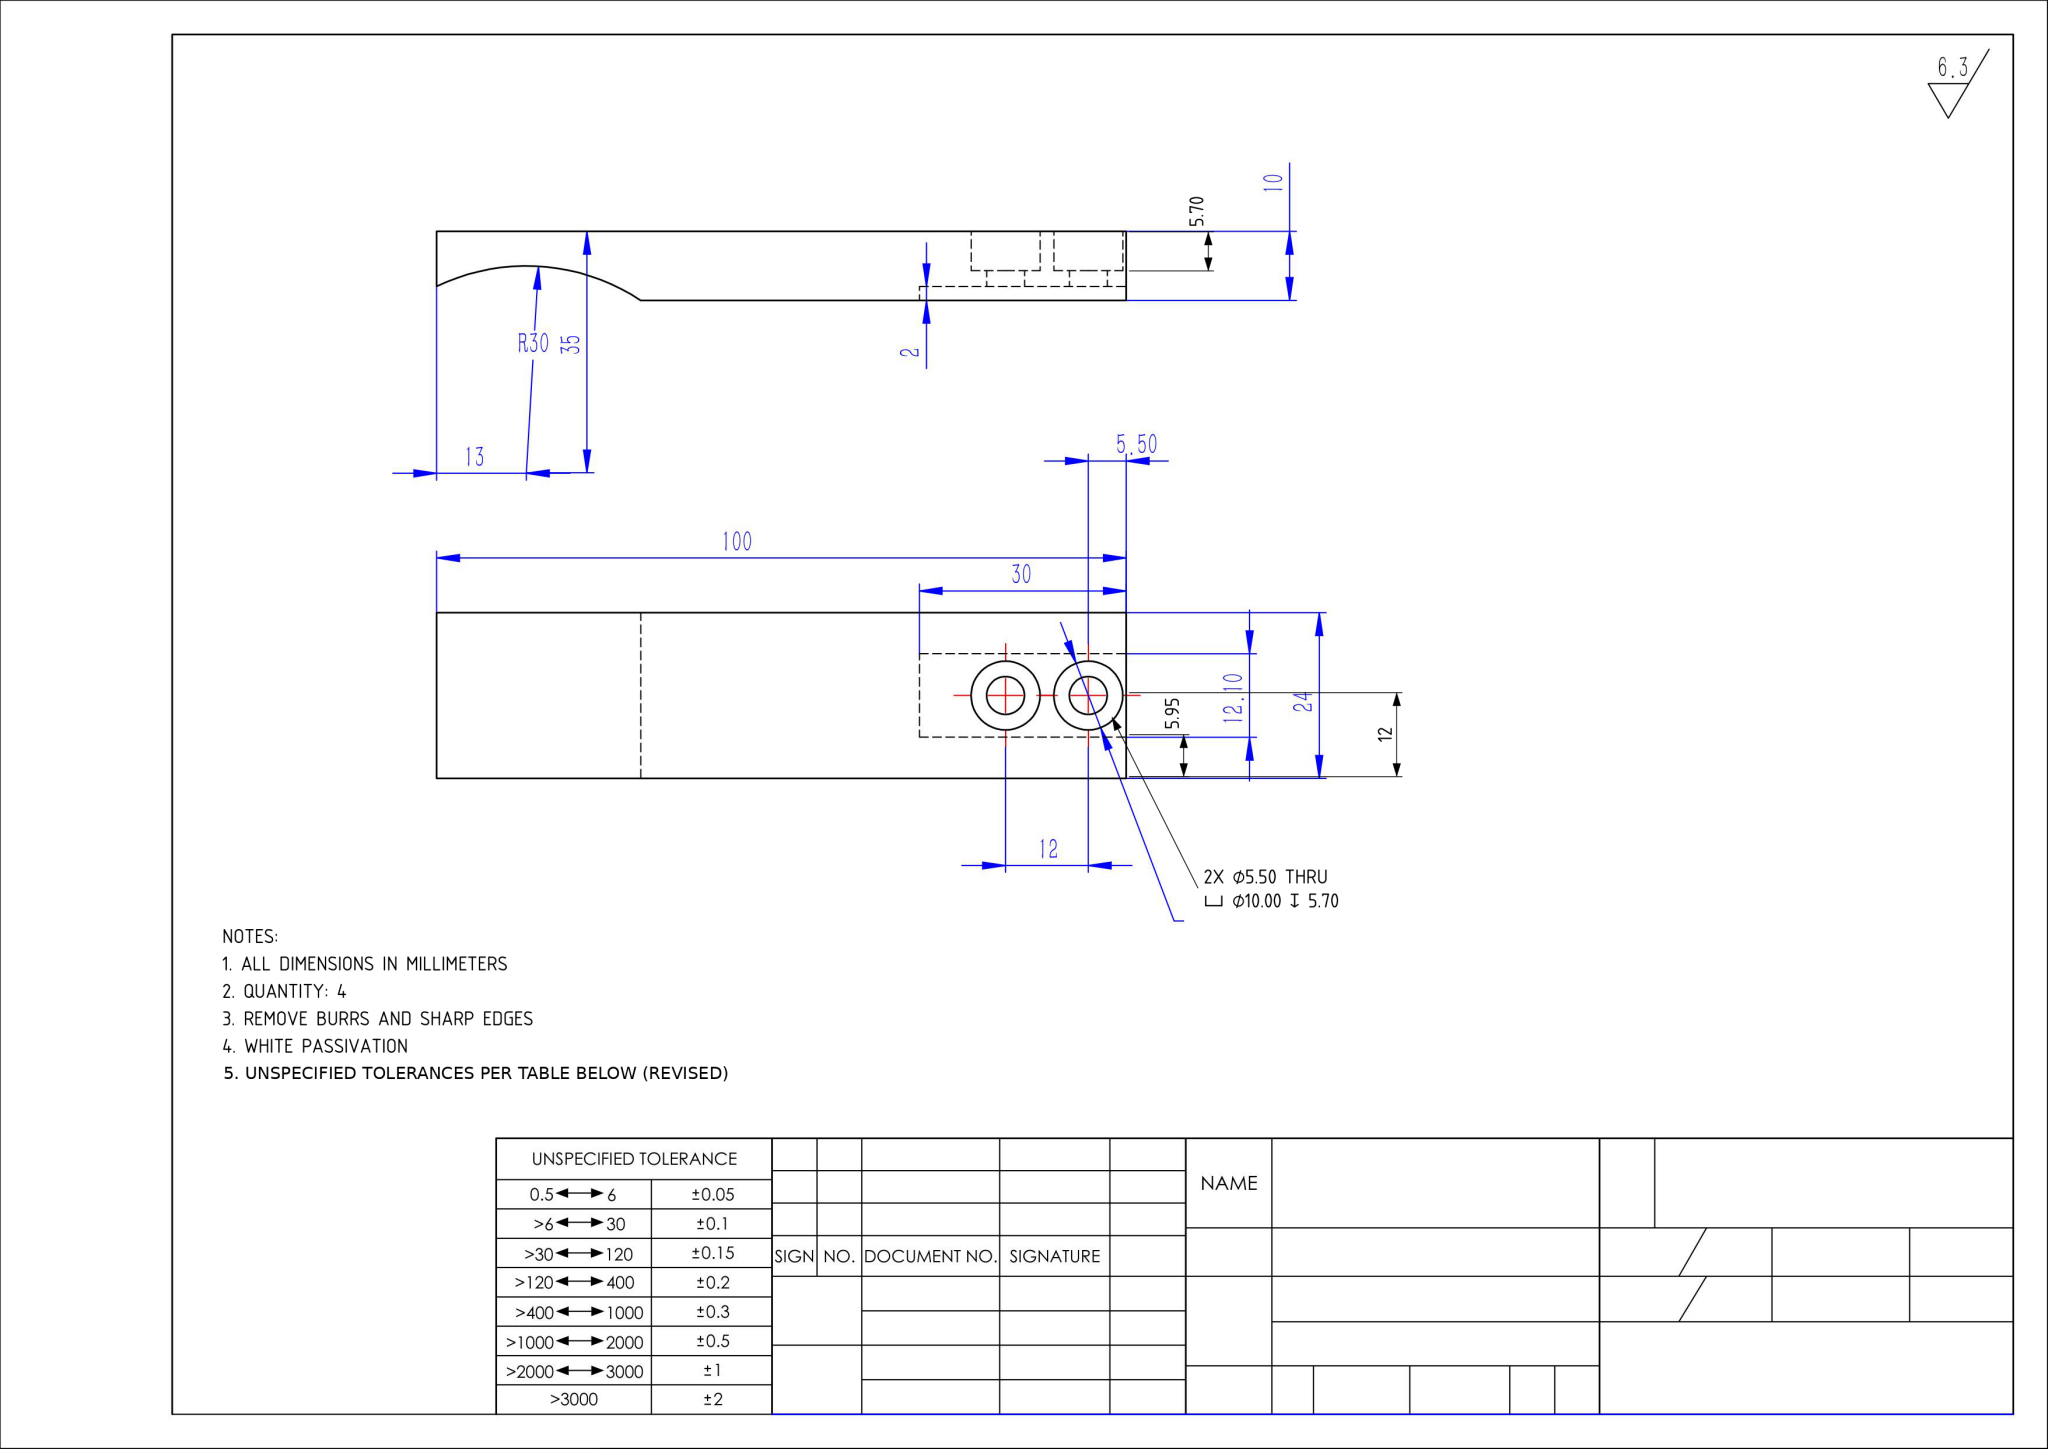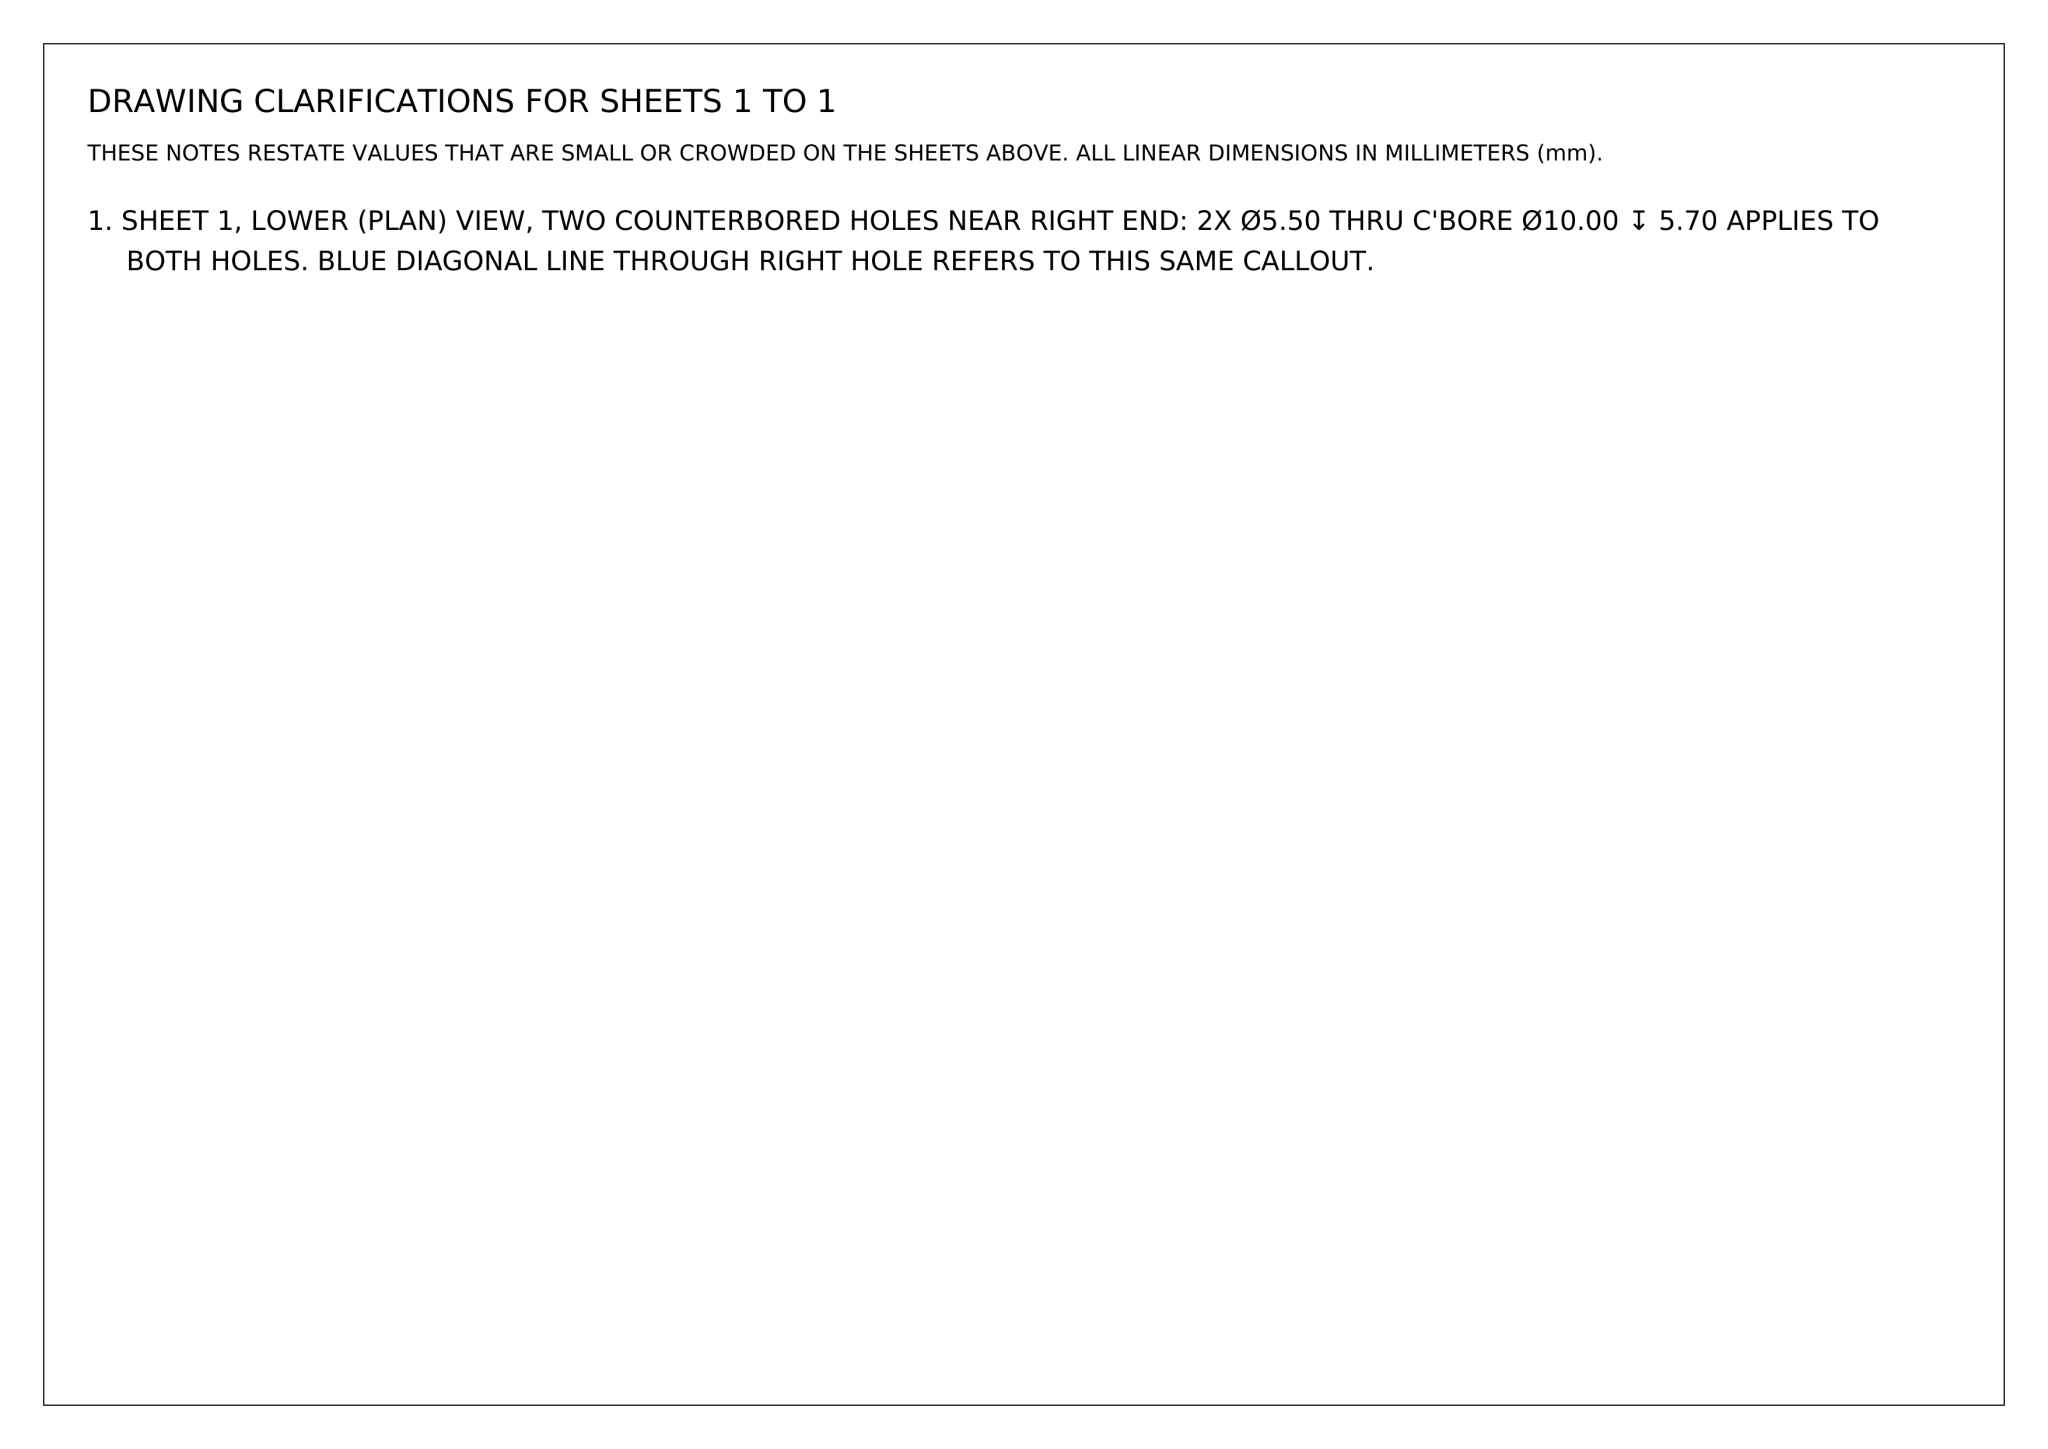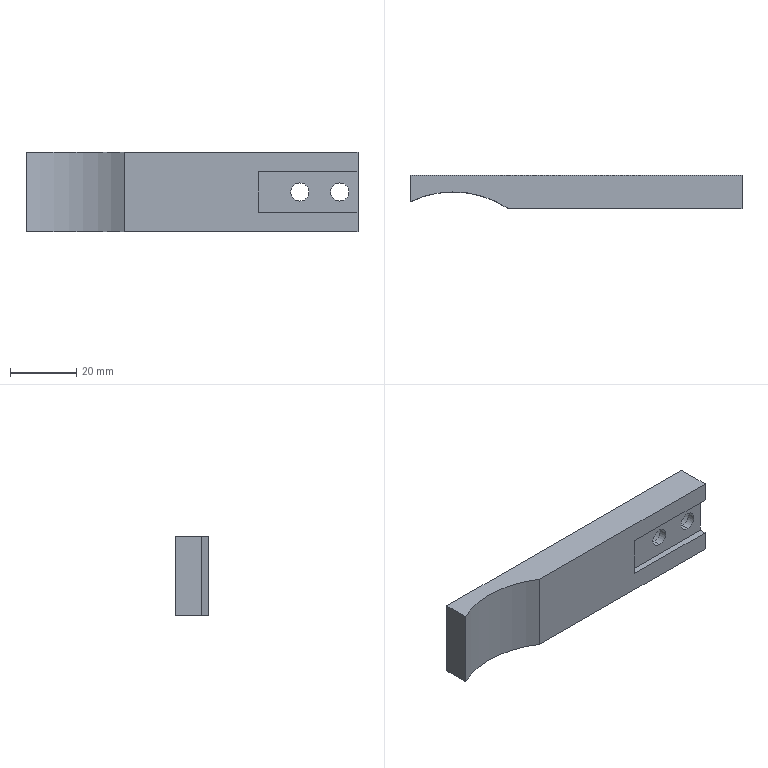Part | NX | mm | Curved End Dual-Bore Mounting Bar | 1 solid | 21 faces | box 100 x 10 x 24 mm | volume 19661 mm3 | plane 12 | cylinder 9 | commonest cylinder face diameters 10 x4 5.5 x4 60 x1
STEP:
#1=COLOUR_RGB('',0.6471,0.5176,0.);
#2=FILL_AREA_STYLE_COLOUR('',#1);
#3=FILL_AREA_STYLE('',(#2));
#4=SURFACE_STYLE_FILL_AREA(#3);
#5=SURFACE_SIDE_STYLE('',(#4));
#6=SURFACE_STYLE_USAGE(.BOTH.,#5);
#7=PRESENTATION_STYLE_ASSIGNMENT((#6));
#8=CARTESIAN_POINT('',(32.5,4.3,-5.));
#9=VERTEX_POINT('',#8);
#10=CARTESIAN_POINT('',(32.5,4.3,5.));
#11=VERTEX_POINT('',#10);
#12=CARTESIAN_POINT('',(32.5,4.3,0.));
#13=DIRECTION('',(0.,1.,0.));
#14=DIRECTION('',(0.,0.,1.));
#15=AXIS2_PLACEMENT_3D('',#12,#13,#14);
#16=CIRCLE('',#15,5.);
#17=EDGE_CURVE('',#9,#11,#16,.T.);
#18=ORIENTED_EDGE('',*,*,#17,.F.);
#19=CARTESIAN_POINT('',(32.5,10.,-5.));
#20=VERTEX_POINT('',#19);
#21=CARTESIAN_POINT('',(32.5,10.,-5.));
#22=DIRECTION('',(0.,1.,0.));
#23=VECTOR('',#22,1000.);
#24=LINE('',#21,#23);
#25=EDGE_CURVE('',#9,#20,#24,.T.);
#26=ORIENTED_EDGE('',*,*,#25,.T.);
#27=CARTESIAN_POINT('',(32.5,10.,5.));
#28=VERTEX_POINT('',#27);
#29=CARTESIAN_POINT('',(32.5,10.,0.));
#30=DIRECTION('',(0.,1.,0.));
#31=DIRECTION('',(0.,0.,1.));
#32=AXIS2_PLACEMENT_3D('',#29,#30,#31);
#33=CIRCLE('',#32,5.);
#34=EDGE_CURVE('',#20,#28,#33,.T.);
#35=ORIENTED_EDGE('',*,*,#34,.T.);
#36=CARTESIAN_POINT('',(32.5,10.,5.));
#37=DIRECTION('',(0.,1.,0.));
#38=VECTOR('',#37,1000.);
#39=LINE('',#36,#38);
#40=EDGE_CURVE('',#11,#28,#39,.T.);
#41=ORIENTED_EDGE('',*,*,#40,.F.);
#42=EDGE_LOOP('',(#18,#26,#35,#41));
#43=FACE_OUTER_BOUND('',#42,.T.);
#44=CARTESIAN_POINT('',(32.5,10.,0.));
#45=DIRECTION('',(0.,1.,0.));
#46=DIRECTION('',(0.,0.,1.));
#47=AXIS2_PLACEMENT_3D('',#44,#45,#46);
#48=CYLINDRICAL_SURFACE('',#47,5.);
#49=ADVANCED_FACE('',(#43),#48,.F.);
#50=CARTESIAN_POINT('',(32.5,2.,2.75));
#51=VERTEX_POINT('',#50);
#52=CARTESIAN_POINT('',(32.5,2.,-2.75));
#53=VERTEX_POINT('',#52);
#54=CARTESIAN_POINT('',(32.5,2.,0.));
#55=DIRECTION('',(0.,-1.,0.));
#56=DIRECTION('',(0.,0.,1.));
#57=AXIS2_PLACEMENT_3D('',#54,#55,#56);
#58=CIRCLE('',#57,2.75);
#59=EDGE_CURVE('',#51,#53,#58,.T.);
#60=ORIENTED_EDGE('',*,*,#59,.T.);
#61=CARTESIAN_POINT('',(32.5,4.3,-2.75));
#62=VERTEX_POINT('',#61);
#63=CARTESIAN_POINT('',(32.5,10.,-2.75));
#64=DIRECTION('',(0.,1.,0.));
#65=VECTOR('',#64,1000.);
#66=LINE('',#63,#65);
#67=EDGE_CURVE('',#53,#62,#66,.T.);
#68=ORIENTED_EDGE('',*,*,#67,.T.);
#69=CARTESIAN_POINT('',(32.5,4.3,2.75));
#70=VERTEX_POINT('',#69);
#71=CARTESIAN_POINT('',(32.5,4.3,0.));
#72=DIRECTION('',(0.,1.,0.));
#73=DIRECTION('',(0.,0.,1.));
#74=AXIS2_PLACEMENT_3D('',#71,#72,#73);
#75=CIRCLE('',#74,2.75);
#76=EDGE_CURVE('',#62,#70,#75,.T.);
#77=ORIENTED_EDGE('',*,*,#76,.T.);
#78=CARTESIAN_POINT('',(32.5,10.,2.75));
#79=DIRECTION('',(0.,1.,0.));
#80=VECTOR('',#79,1000.);
#81=LINE('',#78,#80);
#82=EDGE_CURVE('',#51,#70,#81,.T.);
#83=ORIENTED_EDGE('',*,*,#82,.F.);
#84=EDGE_LOOP('',(#60,#68,#77,#83));
#85=FACE_OUTER_BOUND('',#84,.T.);
#86=CARTESIAN_POINT('',(32.5,10.,0.));
#87=DIRECTION('',(0.,1.,0.));
#88=DIRECTION('',(0.,0.,1.));
#89=AXIS2_PLACEMENT_3D('',#86,#87,#88);
#90=CYLINDRICAL_SURFACE('',#89,2.75);
#91=ADVANCED_FACE('',(#85),#90,.F.);
#92=CARTESIAN_POINT('',(44.5,4.3,-5.));
#93=VERTEX_POINT('',#92);
#94=CARTESIAN_POINT('',(44.5,4.3,5.));
#95=VERTEX_POINT('',#94);
#96=CARTESIAN_POINT('',(44.5,4.3,0.));
#97=DIRECTION('',(0.,1.,0.));
#98=DIRECTION('',(0.,0.,1.));
#99=AXIS2_PLACEMENT_3D('',#96,#97,#98);
#100=CIRCLE('',#99,5.);
#101=EDGE_CURVE('',#93,#95,#100,.T.);
#102=ORIENTED_EDGE('',*,*,#101,.F.);
#103=CARTESIAN_POINT('',(44.5,10.,-5.));
#104=VERTEX_POINT('',#103);
#105=CARTESIAN_POINT('',(44.5,10.,-5.));
#106=DIRECTION('',(0.,1.,0.));
#107=VECTOR('',#106,1000.);
#108=LINE('',#105,#107);
#109=EDGE_CURVE('',#93,#104,#108,.T.);
#110=ORIENTED_EDGE('',*,*,#109,.T.);
#111=CARTESIAN_POINT('',(44.5,10.,5.));
#112=VERTEX_POINT('',#111);
#113=CARTESIAN_POINT('',(44.5,10.,0.));
#114=DIRECTION('',(0.,1.,0.));
#115=DIRECTION('',(0.,0.,1.));
#116=AXIS2_PLACEMENT_3D('',#113,#114,#115);
#117=CIRCLE('',#116,5.);
#118=EDGE_CURVE('',#104,#112,#117,.T.);
#119=ORIENTED_EDGE('',*,*,#118,.T.);
#120=CARTESIAN_POINT('',(44.5,10.,5.));
#121=DIRECTION('',(0.,1.,0.));
#122=VECTOR('',#121,1000.);
#123=LINE('',#120,#122);
#124=EDGE_CURVE('',#95,#112,#123,.T.);
#125=ORIENTED_EDGE('',*,*,#124,.F.);
#126=EDGE_LOOP('',(#102,#110,#119,#125));
#127=FACE_OUTER_BOUND('',#126,.T.);
#128=CARTESIAN_POINT('',(44.5,10.,0.));
#129=DIRECTION('',(0.,1.,0.));
#130=DIRECTION('',(0.,0.,1.));
#131=AXIS2_PLACEMENT_3D('',#128,#129,#130);
#132=CYLINDRICAL_SURFACE('',#131,5.);
#133=ADVANCED_FACE('',(#127),#132,.F.);
#134=CARTESIAN_POINT('',(44.5,2.,2.75));
#135=VERTEX_POINT('',#134);
#136=CARTESIAN_POINT('',(44.5,2.,-2.75));
#137=VERTEX_POINT('',#136);
#138=CARTESIAN_POINT('',(44.5,2.,0.));
#139=DIRECTION('',(0.,-1.,0.));
#140=DIRECTION('',(0.,0.,1.));
#141=AXIS2_PLACEMENT_3D('',#138,#139,#140);
#142=CIRCLE('',#141,2.75);
#143=EDGE_CURVE('',#135,#137,#142,.T.);
#144=ORIENTED_EDGE('',*,*,#143,.T.);
#145=CARTESIAN_POINT('',(44.5,4.3,-2.75));
#146=VERTEX_POINT('',#145);
#147=CARTESIAN_POINT('',(44.5,10.,-2.75));
#148=DIRECTION('',(0.,1.,0.));
#149=VECTOR('',#148,1000.);
#150=LINE('',#147,#149);
#151=EDGE_CURVE('',#137,#146,#150,.T.);
#152=ORIENTED_EDGE('',*,*,#151,.T.);
#153=CARTESIAN_POINT('',(44.5,4.3,2.75));
#154=VERTEX_POINT('',#153);
#155=CARTESIAN_POINT('',(44.5,4.3,0.));
#156=DIRECTION('',(0.,1.,0.));
#157=DIRECTION('',(0.,0.,1.));
#158=AXIS2_PLACEMENT_3D('',#155,#156,#157);
#159=CIRCLE('',#158,2.75);
#160=EDGE_CURVE('',#146,#154,#159,.T.);
#161=ORIENTED_EDGE('',*,*,#160,.T.);
#162=CARTESIAN_POINT('',(44.5,10.,2.75));
#163=DIRECTION('',(0.,1.,0.));
#164=VECTOR('',#163,1000.);
#165=LINE('',#162,#164);
#166=EDGE_CURVE('',#135,#154,#165,.T.);
#167=ORIENTED_EDGE('',*,*,#166,.F.);
#168=EDGE_LOOP('',(#144,#152,#161,#167));
#169=FACE_OUTER_BOUND('',#168,.T.);
#170=CARTESIAN_POINT('',(44.5,10.,0.));
#171=DIRECTION('',(0.,1.,0.));
#172=DIRECTION('',(0.,0.,1.));
#173=AXIS2_PLACEMENT_3D('',#170,#171,#172);
#174=CYLINDRICAL_SURFACE('',#173,2.75);
#175=ADVANCED_FACE('',(#169),#174,.F.);
#176=CARTESIAN_POINT('',(50.,2.,-6.05));
#177=VERTEX_POINT('',#176);
#178=CARTESIAN_POINT('',(50.,2.,6.05));
#179=VERTEX_POINT('',#178);
#180=CARTESIAN_POINT('',(50.,2.,6.05));
#181=DIRECTION('',(0.,0.,1.));
#182=VECTOR('',#181,1000.);
#183=LINE('',#180,#182);
#184=EDGE_CURVE('',#177,#179,#183,.T.);
#185=ORIENTED_EDGE('',*,*,#184,.F.);
#186=CARTESIAN_POINT('',(50.,0.,-6.05));
#187=VERTEX_POINT('',#186);
#188=CARTESIAN_POINT('',(50.,-2.,-6.05));
#189=DIRECTION('',(0.,1.,0.));
#190=VECTOR('',#189,1000.);
#191=LINE('',#188,#190);
#192=EDGE_CURVE('',#187,#177,#191,.T.);
#193=ORIENTED_EDGE('',*,*,#192,.F.);
#194=CARTESIAN_POINT('',(50.,0.,-12.));
#195=VERTEX_POINT('',#194);
#196=CARTESIAN_POINT('',(50.,0.,-12.));
#197=DIRECTION('',(-0.,0.,-1.));
#198=VECTOR('',#197,1000.);
#199=LINE('',#196,#198);
#200=EDGE_CURVE('',#187,#195,#199,.T.);
#201=ORIENTED_EDGE('',*,*,#200,.T.);
#202=CARTESIAN_POINT('',(50.,10.,-12.));
#203=VERTEX_POINT('',#202);
#204=CARTESIAN_POINT('',(50.,10.,-12.));
#205=DIRECTION('',(0.,-1.,0.));
#206=VECTOR('',#205,1000.);
#207=LINE('',#204,#206);
#208=EDGE_CURVE('',#203,#195,#207,.T.);
#209=ORIENTED_EDGE('',*,*,#208,.F.);
#210=CARTESIAN_POINT('',(50.,10.,12.));
#211=VERTEX_POINT('',#210);
#212=CARTESIAN_POINT('',(50.,10.,-12.));
#213=DIRECTION('',(-0.,0.,-1.));
#214=VECTOR('',#213,1000.);
#215=LINE('',#212,#214);
#216=EDGE_CURVE('',#211,#203,#215,.T.);
#217=ORIENTED_EDGE('',*,*,#216,.F.);
#218=CARTESIAN_POINT('',(50.,0.,12.));
#219=VERTEX_POINT('',#218);
#220=CARTESIAN_POINT('',(50.,10.,12.));
#221=DIRECTION('',(0.,-1.,0.));
#222=VECTOR('',#221,1000.);
#223=LINE('',#220,#222);
#224=EDGE_CURVE('',#211,#219,#223,.T.);
#225=ORIENTED_EDGE('',*,*,#224,.T.);
#226=CARTESIAN_POINT('',(50.,0.,6.05));
#227=VERTEX_POINT('',#226);
#228=CARTESIAN_POINT('',(50.,0.,-12.));
#229=DIRECTION('',(-0.,0.,-1.));
#230=VECTOR('',#229,1000.);
#231=LINE('',#228,#230);
#232=EDGE_CURVE('',#219,#227,#231,.T.);
#233=ORIENTED_EDGE('',*,*,#232,.T.);
#234=CARTESIAN_POINT('',(50.,-2.,6.05));
#235=DIRECTION('',(0.,-1.,0.));
#236=VECTOR('',#235,1000.);
#237=LINE('',#234,#236);
#238=EDGE_CURVE('',#179,#227,#237,.T.);
#239=ORIENTED_EDGE('',*,*,#238,.F.);
#240=EDGE_LOOP('',(#185,#193,#201,#209,#217,#225,#233,#239));
#241=FACE_OUTER_BOUND('',#240,.T.);
#242=CARTESIAN_POINT('',(50.,10.,-12.));
#243=DIRECTION('',(-1.,0.,0.));
#244=DIRECTION('',(0.,0.,1.));
#245=AXIS2_PLACEMENT_3D('',#242,#243,#244);
#246=PLANE('',#245);
#247=ADVANCED_FACE('',(#241),#246,.F.);
#248=CARTESIAN_POINT('',(-20.417,0.,-12.));
#249=VERTEX_POINT('',#248);
#250=CARTESIAN_POINT('',(-50.,0.,-12.));
#251=DIRECTION('',(-1.,0.,0.));
#252=VECTOR('',#251,1000.);
#253=LINE('',#250,#252);
#254=EDGE_CURVE('',#195,#249,#253,.T.);
#255=ORIENTED_EDGE('',*,*,#254,.T.);
#256=CARTESIAN_POINT('',(-50.,2.037,-12.));
#257=VERTEX_POINT('',#256);
#258=CARTESIAN_POINT('',(-37.,-25.,-12.));
#259=DIRECTION('',(0.,0.,-1.));
#260=DIRECTION('',(-1.,0.,0.));
#261=AXIS2_PLACEMENT_3D('',#258,#259,#260);
#262=CIRCLE('',#261,30.);
#263=EDGE_CURVE('',#257,#249,#262,.T.);
#264=ORIENTED_EDGE('',*,*,#263,.F.);
#265=CARTESIAN_POINT('',(-50.,10.,-12.));
#266=VERTEX_POINT('',#265);
#267=CARTESIAN_POINT('',(-50.,10.,-12.));
#268=DIRECTION('',(0.,-1.,0.));
#269=VECTOR('',#268,1000.);
#270=LINE('',#267,#269);
#271=EDGE_CURVE('',#266,#257,#270,.T.);
#272=ORIENTED_EDGE('',*,*,#271,.F.);
#273=CARTESIAN_POINT('',(-50.,10.,-12.));
#274=DIRECTION('',(-1.,0.,0.));
#275=VECTOR('',#274,1000.);
#276=LINE('',#273,#275);
#277=EDGE_CURVE('',#203,#266,#276,.T.);
#278=ORIENTED_EDGE('',*,*,#277,.F.);
#279=ORIENTED_EDGE('',*,*,#208,.T.);
#280=EDGE_LOOP('',(#255,#264,#272,#278,#279));
#281=FACE_OUTER_BOUND('',#280,.T.);
#282=CARTESIAN_POINT('',(-50.,10.,-12.));
#283=DIRECTION('',(0.,0.,1.));
#284=DIRECTION('',(1.,0.,0.));
#285=AXIS2_PLACEMENT_3D('',#282,#283,#284);
#286=PLANE('',#285);
#287=ADVANCED_FACE('',(#281),#286,.F.);
#288=ORIENTED_EDGE('',*,*,#271,.T.);
#289=CARTESIAN_POINT('',(-50.,2.037,12.));
#290=VERTEX_POINT('',#289);
#291=CARTESIAN_POINT('',(-50.,2.037,12.));
#292=DIRECTION('',(0.,0.,1.));
#293=VECTOR('',#292,1000.);
#294=LINE('',#291,#293);
#295=EDGE_CURVE('',#257,#290,#294,.T.);
#296=ORIENTED_EDGE('',*,*,#295,.T.);
#297=CARTESIAN_POINT('',(-50.,10.,12.));
#298=VERTEX_POINT('',#297);
#299=CARTESIAN_POINT('',(-50.,10.,12.));
#300=DIRECTION('',(0.,-1.,0.));
#301=VECTOR('',#300,1000.);
#302=LINE('',#299,#301);
#303=EDGE_CURVE('',#298,#290,#302,.T.);
#304=ORIENTED_EDGE('',*,*,#303,.F.);
#305=CARTESIAN_POINT('',(-50.,10.,-12.));
#306=DIRECTION('',(-0.,0.,1.));
#307=VECTOR('',#306,1000.);
#308=LINE('',#305,#307);
#309=EDGE_CURVE('',#266,#298,#308,.T.);
#310=ORIENTED_EDGE('',*,*,#309,.F.);
#311=EDGE_LOOP('',(#288,#296,#304,#310));
#312=FACE_OUTER_BOUND('',#311,.T.);
#313=CARTESIAN_POINT('',(-50.,10.,-12.));
#314=DIRECTION('',(1.,0.,0.));
#315=DIRECTION('',(0.,0.,-1.));
#316=AXIS2_PLACEMENT_3D('',#313,#314,#315);
#317=PLANE('',#316);
#318=ADVANCED_FACE('',(#312),#317,.F.);
#319=ORIENTED_EDGE('',*,*,#303,.T.);
#320=CARTESIAN_POINT('',(-20.417,0.,12.));
#321=VERTEX_POINT('',#320);
#322=CARTESIAN_POINT('',(-37.,-25.,12.));
#323=DIRECTION('',(0.,0.,-1.));
#324=DIRECTION('',(-1.,0.,0.));
#325=AXIS2_PLACEMENT_3D('',#322,#323,#324);
#326=CIRCLE('',#325,30.);
#327=EDGE_CURVE('',#290,#321,#326,.T.);
#328=ORIENTED_EDGE('',*,*,#327,.T.);
#329=CARTESIAN_POINT('',(-50.,0.,12.));
#330=DIRECTION('',(1.,0.,0.));
#331=VECTOR('',#330,1000.);
#332=LINE('',#329,#331);
#333=EDGE_CURVE('',#321,#219,#332,.T.);
#334=ORIENTED_EDGE('',*,*,#333,.T.);
#335=ORIENTED_EDGE('',*,*,#224,.F.);
#336=CARTESIAN_POINT('',(-50.,10.,12.));
#337=DIRECTION('',(1.,0.,0.));
#338=VECTOR('',#337,1000.);
#339=LINE('',#336,#338);
#340=EDGE_CURVE('',#298,#211,#339,.T.);
#341=ORIENTED_EDGE('',*,*,#340,.F.);
#342=EDGE_LOOP('',(#319,#328,#334,#335,#341));
#343=FACE_OUTER_BOUND('',#342,.T.);
#344=CARTESIAN_POINT('',(-50.,10.,12.));
#345=DIRECTION('',(0.,0.,-1.));
#346=DIRECTION('',(-1.,0.,0.));
#347=AXIS2_PLACEMENT_3D('',#344,#345,#346);
#348=PLANE('',#347);
#349=ADVANCED_FACE('',(#343),#348,.F.);
#350=CARTESIAN_POINT('',(32.5,10.,0.));
#351=DIRECTION('',(0.,1.,0.));
#352=DIRECTION('',(0.,0.,1.));
#353=AXIS2_PLACEMENT_3D('',#350,#351,#352);
#354=CIRCLE('',#353,5.);
#355=EDGE_CURVE('',#28,#20,#354,.T.);
#356=ORIENTED_EDGE('',*,*,#355,.F.);
#357=ORIENTED_EDGE('',*,*,#34,.F.);
#358=EDGE_LOOP('',(#356,#357));
#359=FACE_BOUND('',#358,.T.);
#360=CARTESIAN_POINT('',(44.5,10.,0.));
#361=DIRECTION('',(0.,1.,0.));
#362=DIRECTION('',(0.,0.,1.));
#363=AXIS2_PLACEMENT_3D('',#360,#361,#362);
#364=CIRCLE('',#363,5.);
#365=EDGE_CURVE('',#112,#104,#364,.T.);
#366=ORIENTED_EDGE('',*,*,#365,.F.);
#367=ORIENTED_EDGE('',*,*,#118,.F.);
#368=EDGE_LOOP('',(#366,#367));
#369=FACE_BOUND('',#368,.T.);
#370=ORIENTED_EDGE('',*,*,#216,.T.);
#371=ORIENTED_EDGE('',*,*,#277,.T.);
#372=ORIENTED_EDGE('',*,*,#309,.T.);
#373=ORIENTED_EDGE('',*,*,#340,.T.);
#374=EDGE_LOOP('',(#370,#371,#372,#373));
#375=FACE_OUTER_BOUND('',#374,.T.);
#376=CARTESIAN_POINT('',(0.,10.,0.));
#377=DIRECTION('',(0.,1.,0.));
#378=DIRECTION('',(0.,0.,1.));
#379=AXIS2_PLACEMENT_3D('',#376,#377,#378);
#380=PLANE('',#379);
#381=ADVANCED_FACE('',(#359,#369,#375),#380,.T.);
#382=ORIENTED_EDGE('',*,*,#333,.F.);
#383=CARTESIAN_POINT('',(-20.417,0.,12.));
#384=DIRECTION('',(0.,0.,-1.));
#385=VECTOR('',#384,1000.);
#386=LINE('',#383,#385);
#387=EDGE_CURVE('',#321,#249,#386,.T.);
#388=ORIENTED_EDGE('',*,*,#387,.T.);
#389=ORIENTED_EDGE('',*,*,#254,.F.);
#390=ORIENTED_EDGE('',*,*,#200,.F.);
#391=CARTESIAN_POINT('',(20.,0.,-6.05));
#392=VERTEX_POINT('',#391);
#393=CARTESIAN_POINT('',(0.,0.,-6.05));
#394=DIRECTION('',(-1.,0.,0.));
#395=VECTOR('',#394,1000.);
#396=LINE('',#393,#395);
#397=EDGE_CURVE('',#187,#392,#396,.T.);
#398=ORIENTED_EDGE('',*,*,#397,.T.);
#399=CARTESIAN_POINT('',(20.,0.,6.05));
#400=VERTEX_POINT('',#399);
#401=CARTESIAN_POINT('',(20.,0.,0.));
#402=DIRECTION('',(0.,0.,1.));
#403=VECTOR('',#402,1000.);
#404=LINE('',#401,#403);
#405=EDGE_CURVE('',#392,#400,#404,.T.);
#406=ORIENTED_EDGE('',*,*,#405,.T.);
#407=CARTESIAN_POINT('',(0.,0.,6.05));
#408=DIRECTION('',(1.,0.,0.));
#409=VECTOR('',#408,1000.);
#410=LINE('',#407,#409);
#411=EDGE_CURVE('',#400,#227,#410,.T.);
#412=ORIENTED_EDGE('',*,*,#411,.T.);
#413=ORIENTED_EDGE('',*,*,#232,.F.);
#414=EDGE_LOOP('',(#382,#388,#389,#390,#398,#406,#412,#413));
#415=FACE_OUTER_BOUND('',#414,.T.);
#416=CARTESIAN_POINT('',(0.,0.,0.));
#417=DIRECTION('',(0.,1.,0.));
#418=DIRECTION('',(0.,0.,1.));
#419=AXIS2_PLACEMENT_3D('',#416,#417,#418);
#420=PLANE('',#419);
#421=ADVANCED_FACE('',(#415),#420,.F.);
#422=ORIENTED_EDGE('',*,*,#151,.F.);
#423=CARTESIAN_POINT('',(44.5,2.,0.));
#424=DIRECTION('',(0.,-1.,0.));
#425=DIRECTION('',(0.,0.,1.));
#426=AXIS2_PLACEMENT_3D('',#423,#424,#425);
#427=CIRCLE('',#426,2.75);
#428=EDGE_CURVE('',#137,#135,#427,.T.);
#429=ORIENTED_EDGE('',*,*,#428,.T.);
#430=ORIENTED_EDGE('',*,*,#166,.T.);
#431=CARTESIAN_POINT('',(44.5,4.3,0.));
#432=DIRECTION('',(0.,1.,0.));
#433=DIRECTION('',(0.,0.,1.));
#434=AXIS2_PLACEMENT_3D('',#431,#432,#433);
#435=CIRCLE('',#434,2.75);
#436=EDGE_CURVE('',#154,#146,#435,.T.);
#437=ORIENTED_EDGE('',*,*,#436,.T.);
#438=EDGE_LOOP('',(#422,#429,#430,#437));
#439=FACE_OUTER_BOUND('',#438,.T.);
#440=CARTESIAN_POINT('',(44.5,10.,0.));
#441=DIRECTION('',(0.,1.,0.));
#442=DIRECTION('',(0.,0.,1.));
#443=AXIS2_PLACEMENT_3D('',#440,#441,#442);
#444=CYLINDRICAL_SURFACE('',#443,2.75);
#445=ADVANCED_FACE('',(#439),#444,.F.);
#446=ORIENTED_EDGE('',*,*,#436,.F.);
#447=ORIENTED_EDGE('',*,*,#160,.F.);
#448=EDGE_LOOP('',(#446,#447));
#449=FACE_BOUND('',#448,.T.);
#450=CARTESIAN_POINT('',(44.5,4.3,0.));
#451=DIRECTION('',(0.,1.,0.));
#452=DIRECTION('',(0.,0.,1.));
#453=AXIS2_PLACEMENT_3D('',#450,#451,#452);
#454=CIRCLE('',#453,5.);
#455=EDGE_CURVE('',#95,#93,#454,.T.);
#456=ORIENTED_EDGE('',*,*,#455,.T.);
#457=ORIENTED_EDGE('',*,*,#101,.T.);
#458=EDGE_LOOP('',(#456,#457));
#459=FACE_OUTER_BOUND('',#458,.T.);
#460=CARTESIAN_POINT('',(47.25,4.3,0.));
#461=DIRECTION('',(0.,-1.,0.));
#462=DIRECTION('',(0.,0.,-1.));
#463=AXIS2_PLACEMENT_3D('',#460,#461,#462);
#464=PLANE('',#463);
#465=ADVANCED_FACE('',(#449,#459),#464,.F.);
#466=ORIENTED_EDGE('',*,*,#109,.F.);
#467=ORIENTED_EDGE('',*,*,#455,.F.);
#468=ORIENTED_EDGE('',*,*,#124,.T.);
#469=ORIENTED_EDGE('',*,*,#365,.T.);
#470=EDGE_LOOP('',(#466,#467,#468,#469));
#471=FACE_OUTER_BOUND('',#470,.T.);
#472=CARTESIAN_POINT('',(44.5,10.,0.));
#473=DIRECTION('',(0.,1.,0.));
#474=DIRECTION('',(0.,0.,1.));
#475=AXIS2_PLACEMENT_3D('',#472,#473,#474);
#476=CYLINDRICAL_SURFACE('',#475,5.);
#477=ADVANCED_FACE('',(#471),#476,.F.);
#478=ORIENTED_EDGE('',*,*,#67,.F.);
#479=CARTESIAN_POINT('',(32.5,2.,0.));
#480=DIRECTION('',(0.,-1.,0.));
#481=DIRECTION('',(0.,0.,1.));
#482=AXIS2_PLACEMENT_3D('',#479,#480,#481);
#483=CIRCLE('',#482,2.75);
#484=EDGE_CURVE('',#53,#51,#483,.T.);
#485=ORIENTED_EDGE('',*,*,#484,.T.);
#486=ORIENTED_EDGE('',*,*,#82,.T.);
#487=CARTESIAN_POINT('',(32.5,4.3,0.));
#488=DIRECTION('',(0.,1.,0.));
#489=DIRECTION('',(0.,0.,1.));
#490=AXIS2_PLACEMENT_3D('',#487,#488,#489);
#491=CIRCLE('',#490,2.75);
#492=EDGE_CURVE('',#70,#62,#491,.T.);
#493=ORIENTED_EDGE('',*,*,#492,.T.);
#494=EDGE_LOOP('',(#478,#485,#486,#493));
#495=FACE_OUTER_BOUND('',#494,.T.);
#496=CARTESIAN_POINT('',(32.5,10.,0.));
#497=DIRECTION('',(0.,1.,0.));
#498=DIRECTION('',(0.,0.,1.));
#499=AXIS2_PLACEMENT_3D('',#496,#497,#498);
#500=CYLINDRICAL_SURFACE('',#499,2.75);
#501=ADVANCED_FACE('',(#495),#500,.F.);
#502=ORIENTED_EDGE('',*,*,#492,.F.);
#503=ORIENTED_EDGE('',*,*,#76,.F.);
#504=EDGE_LOOP('',(#502,#503));
#505=FACE_BOUND('',#504,.T.);
#506=CARTESIAN_POINT('',(32.5,4.3,0.));
#507=DIRECTION('',(0.,1.,0.));
#508=DIRECTION('',(0.,0.,1.));
#509=AXIS2_PLACEMENT_3D('',#506,#507,#508);
#510=CIRCLE('',#509,5.);
#511=EDGE_CURVE('',#11,#9,#510,.T.);
#512=ORIENTED_EDGE('',*,*,#511,.T.);
#513=ORIENTED_EDGE('',*,*,#17,.T.);
#514=EDGE_LOOP('',(#512,#513));
#515=FACE_OUTER_BOUND('',#514,.T.);
#516=CARTESIAN_POINT('',(35.25,4.3,0.));
#517=DIRECTION('',(0.,-1.,0.));
#518=DIRECTION('',(0.,0.,-1.));
#519=AXIS2_PLACEMENT_3D('',#516,#517,#518);
#520=PLANE('',#519);
#521=ADVANCED_FACE('',(#505,#515),#520,.F.);
#522=ORIENTED_EDGE('',*,*,#25,.F.);
#523=ORIENTED_EDGE('',*,*,#511,.F.);
#524=ORIENTED_EDGE('',*,*,#40,.T.);
#525=ORIENTED_EDGE('',*,*,#355,.T.);
#526=EDGE_LOOP('',(#522,#523,#524,#525));
#527=FACE_OUTER_BOUND('',#526,.T.);
#528=CARTESIAN_POINT('',(32.5,10.,0.));
#529=DIRECTION('',(0.,1.,0.));
#530=DIRECTION('',(0.,0.,1.));
#531=AXIS2_PLACEMENT_3D('',#528,#529,#530);
#532=CYLINDRICAL_SURFACE('',#531,5.);
#533=ADVANCED_FACE('',(#527),#532,.F.);
#534=ORIENTED_EDGE('',*,*,#192,.T.);
#535=CARTESIAN_POINT('',(20.,2.,-6.05));
#536=VERTEX_POINT('',#535);
#537=CARTESIAN_POINT('',(20.,2.,-6.05));
#538=DIRECTION('',(1.,0.,0.));
#539=VECTOR('',#538,1000.);
#540=LINE('',#537,#539);
#541=EDGE_CURVE('',#536,#177,#540,.T.);
#542=ORIENTED_EDGE('',*,*,#541,.F.);
#543=CARTESIAN_POINT('',(20.,-2.,-6.05));
#544=DIRECTION('',(0.,1.,0.));
#545=VECTOR('',#544,1000.);
#546=LINE('',#543,#545);
#547=EDGE_CURVE('',#392,#536,#546,.T.);
#548=ORIENTED_EDGE('',*,*,#547,.F.);
#549=ORIENTED_EDGE('',*,*,#397,.F.);
#550=EDGE_LOOP('',(#534,#542,#548,#549));
#551=FACE_OUTER_BOUND('',#550,.T.);
#552=CARTESIAN_POINT('',(20.,-2.,-6.05));
#553=DIRECTION('',(0.,0.,-1.));
#554=DIRECTION('',(-1.,0.,0.));
#555=AXIS2_PLACEMENT_3D('',#552,#553,#554);
#556=PLANE('',#555);
#557=ADVANCED_FACE('',(#551),#556,.F.);
#558=CARTESIAN_POINT('',(20.,2.,6.05));
#559=VERTEX_POINT('',#558);
#560=CARTESIAN_POINT('',(20.,-2.,6.05));
#561=DIRECTION('',(0.,-1.,0.));
#562=VECTOR('',#561,1000.);
#563=LINE('',#560,#562);
#564=EDGE_CURVE('',#559,#400,#563,.T.);
#565=ORIENTED_EDGE('',*,*,#564,.F.);
#566=CARTESIAN_POINT('',(20.,2.,6.05));
#567=DIRECTION('',(1.,0.,0.));
#568=VECTOR('',#567,1000.);
#569=LINE('',#566,#568);
#570=EDGE_CURVE('',#559,#179,#569,.T.);
#571=ORIENTED_EDGE('',*,*,#570,.T.);
#572=ORIENTED_EDGE('',*,*,#238,.T.);
#573=ORIENTED_EDGE('',*,*,#411,.F.);
#574=EDGE_LOOP('',(#565,#571,#572,#573));
#575=FACE_OUTER_BOUND('',#574,.T.);
#576=CARTESIAN_POINT('',(20.,-2.,6.05));
#577=DIRECTION('',(0.,0.,1.));
#578=DIRECTION('',(1.,0.,0.));
#579=AXIS2_PLACEMENT_3D('',#576,#577,#578);
#580=PLANE('',#579);
#581=ADVANCED_FACE('',(#575),#580,.F.);
#582=ORIENTED_EDGE('',*,*,#547,.T.);
#583=CARTESIAN_POINT('',(20.,2.,6.05));
#584=DIRECTION('',(0.,0.,1.));
#585=VECTOR('',#584,1000.);
#586=LINE('',#583,#585);
#587=EDGE_CURVE('',#536,#559,#586,.T.);
#588=ORIENTED_EDGE('',*,*,#587,.T.);
#589=ORIENTED_EDGE('',*,*,#564,.T.);
#590=ORIENTED_EDGE('',*,*,#405,.F.);
#591=EDGE_LOOP('',(#582,#588,#589,#590));
#592=FACE_OUTER_BOUND('',#591,.T.);
#593=CARTESIAN_POINT('',(20.,0.,0.));
#594=DIRECTION('',(-1.,0.,0.));
#595=DIRECTION('',(0.,0.,1.));
#596=AXIS2_PLACEMENT_3D('',#593,#594,#595);
#597=PLANE('',#596);
#598=ADVANCED_FACE('',(#592),#597,.F.);
#599=ORIENTED_EDGE('',*,*,#59,.F.);
#600=ORIENTED_EDGE('',*,*,#484,.F.);
#601=EDGE_LOOP('',(#599,#600));
#602=FACE_BOUND('',#601,.T.);
#603=ORIENTED_EDGE('',*,*,#184,.T.);
#604=ORIENTED_EDGE('',*,*,#570,.F.);
#605=ORIENTED_EDGE('',*,*,#587,.F.);
#606=ORIENTED_EDGE('',*,*,#541,.T.);
#607=EDGE_LOOP('',(#603,#604,#605,#606));
#608=FACE_OUTER_BOUND('',#607,.T.);
#609=ORIENTED_EDGE('',*,*,#143,.F.);
#610=ORIENTED_EDGE('',*,*,#428,.F.);
#611=EDGE_LOOP('',(#609,#610));
#612=FACE_BOUND('',#611,.T.);
#613=CARTESIAN_POINT('',(20.,2.,6.05));
#614=DIRECTION('',(0.,1.,0.));
#615=DIRECTION('',(0.,0.,1.));
#616=AXIS2_PLACEMENT_3D('',#613,#614,#615);
#617=PLANE('',#616);
#618=ADVANCED_FACE('',(#602,#608,#612),#617,.F.);
#619=ORIENTED_EDGE('',*,*,#263,.T.);
#620=ORIENTED_EDGE('',*,*,#387,.F.);
#621=ORIENTED_EDGE('',*,*,#327,.F.);
#622=ORIENTED_EDGE('',*,*,#295,.F.);
#623=EDGE_LOOP('',(#619,#620,#621,#622));
#624=FACE_OUTER_BOUND('',#623,.T.);
#625=CARTESIAN_POINT('',(-37.,-25.,12.));
#626=DIRECTION('',(0.,0.,-1.));
#627=DIRECTION('',(-1.,0.,0.));
#628=AXIS2_PLACEMENT_3D('',#625,#626,#627);
#629=CYLINDRICAL_SURFACE('',#628,30.);
#630=ADVANCED_FACE('',(#624),#629,.F.);
#631=CLOSED_SHELL('',(#49,#91,#133,#175,#247,#287,#318,#349,#381,#421,#445,#465,#477,#501,#521,#533,#557,#581,#598,#618,#630));
#632=MANIFOLD_SOLID_BREP('',#631);
#633=STYLED_ITEM('',(#7),#632);
#634=(LENGTH_UNIT()NAMED_UNIT(*)SI_UNIT(.MILLI.,.METRE.));
#635=UNCERTAINTY_MEASURE_WITH_UNIT(LENGTH_MEASURE(0.00001),#634,'','');
#636=(NAMED_UNIT(*)PLANE_ANGLE_UNIT()SI_UNIT($,.RADIAN.));
#637=(NAMED_UNIT(*)SI_UNIT($,.STERADIAN.)SOLID_ANGLE_UNIT());
#638=(GEOMETRIC_REPRESENTATION_CONTEXT(3)GLOBAL_UNCERTAINTY_ASSIGNED_CONTEXT((#635))GLOBAL_UNIT_ASSIGNED_CONTEXT((#634,#636,#637))REPRESENTATION_CONTEXT('',''));
#639=MECHANICAL_DESIGN_GEOMETRIC_PRESENTATION_REPRESENTATION('',(#633),#638);
#640=COLOUR_RGB('',0.6471,0.5176,0.);
#641=FILL_AREA_STYLE_COLOUR('',#640);
#642=FILL_AREA_STYLE('',(#641));
#643=SURFACE_STYLE_FILL_AREA(#642);
#644=SURFACE_SIDE_STYLE('',(#643));
#645=SURFACE_STYLE_USAGE(.BOTH.,#644);
#646=PRESENTATION_STYLE_ASSIGNMENT((#645));
#647=CARTESIAN_POINT('',(0.,0.,0.));
#648=DIRECTION('',(0.,0.,1.));
#649=DIRECTION('',(1.,0.,0.));
#650=AXIS2_PLACEMENT_3D('',#647,#648,#649);
#651=(LENGTH_UNIT()NAMED_UNIT(*)SI_UNIT(.MILLI.,.METRE.));
#652=UNCERTAINTY_MEASURE_WITH_UNIT(LENGTH_MEASURE(0.00001),#651,'','');
#653=(NAMED_UNIT(*)PLANE_ANGLE_UNIT()SI_UNIT($,.RADIAN.));
#654=(NAMED_UNIT(*)SI_UNIT($,.STERADIAN.)SOLID_ANGLE_UNIT());
#655=(GEOMETRIC_REPRESENTATION_CONTEXT(3)GLOBAL_UNCERTAINTY_ASSIGNED_CONTEXT((#652))GLOBAL_UNIT_ASSIGNED_CONTEXT((#651,#653,#654))REPRESENTATION_CONTEXT('',''));
#656=ADVANCED_BREP_SHAPE_REPRESENTATION('',(#632,#650),#655);
#657=STYLED_ITEM('',(#646),#656);
#658=PRESENTATION_LAYER_ASSIGNMENT('','',(#657));
#659=PRESENTATION_LAYER_ASSIGNMENT('','',(#633));
#660=(LENGTH_UNIT()NAMED_UNIT(*)SI_UNIT(.MILLI.,.METRE.));
#661=UNCERTAINTY_MEASURE_WITH_UNIT(LENGTH_MEASURE(0.00001),#660,'','');
#662=(NAMED_UNIT(*)PLANE_ANGLE_UNIT()SI_UNIT($,.RADIAN.));
#663=(NAMED_UNIT(*)SI_UNIT($,.STERADIAN.)SOLID_ANGLE_UNIT());
#664=(GEOMETRIC_REPRESENTATION_CONTEXT(3)GLOBAL_UNCERTAINTY_ASSIGNED_CONTEXT((#661))GLOBAL_UNIT_ASSIGNED_CONTEXT((#660,#662,#663))REPRESENTATION_CONTEXT('',''));
#665=MECHANICAL_DESIGN_GEOMETRIC_PRESENTATION_REPRESENTATION('',(#657),#664);